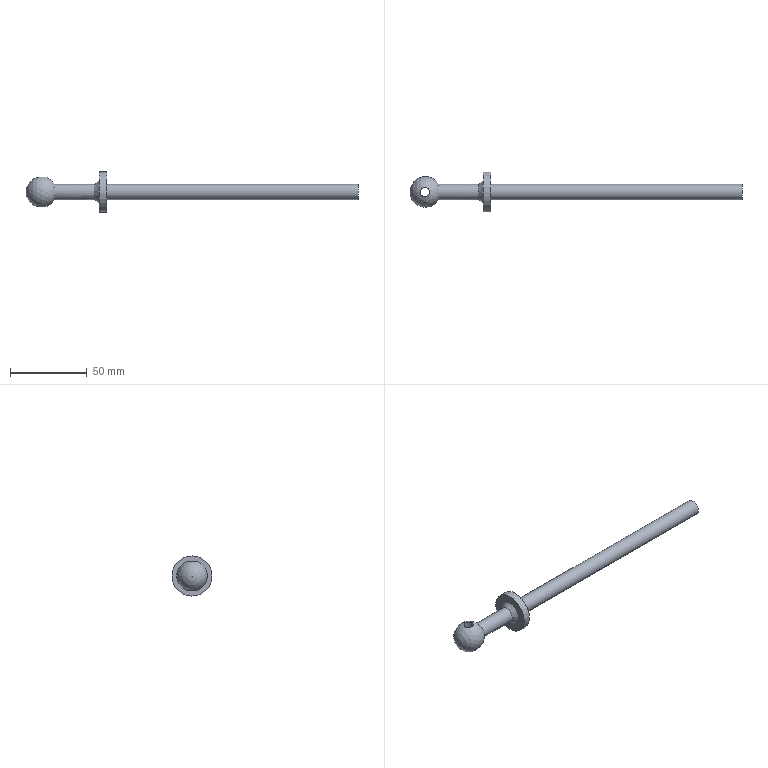Component | NX | MOVING_ROD | 1 solid | 13 faces | volume 21057 mm3 | cylinder 6 | plane 5 | sphere 1 | cone 1 | commonest cylinder face diameters 10 x3 6 x2 26 x1